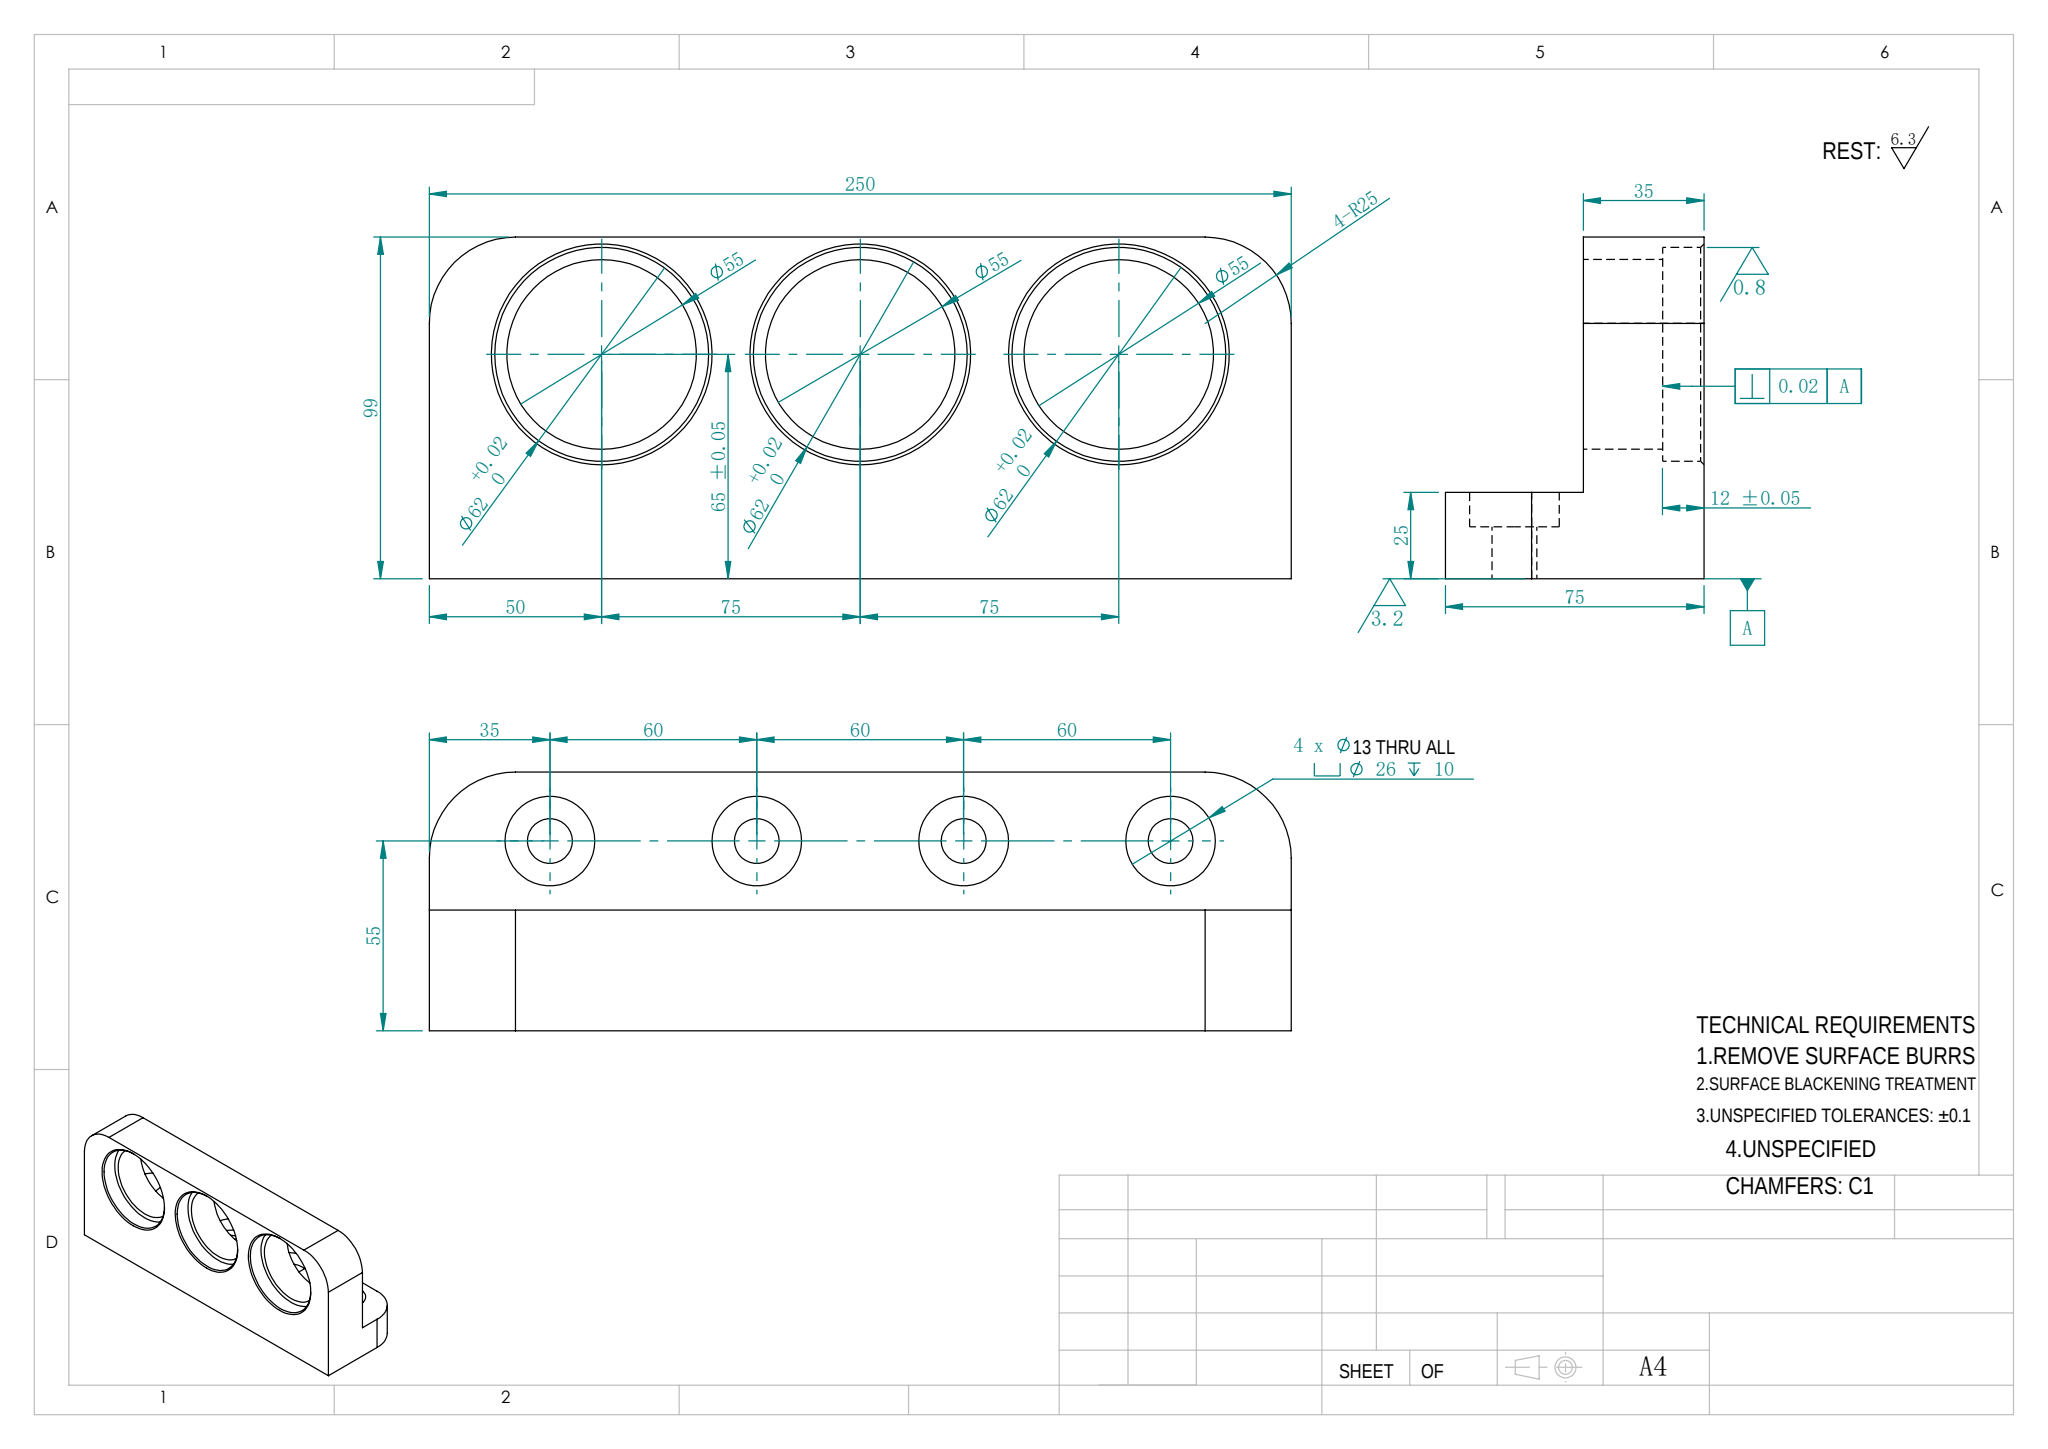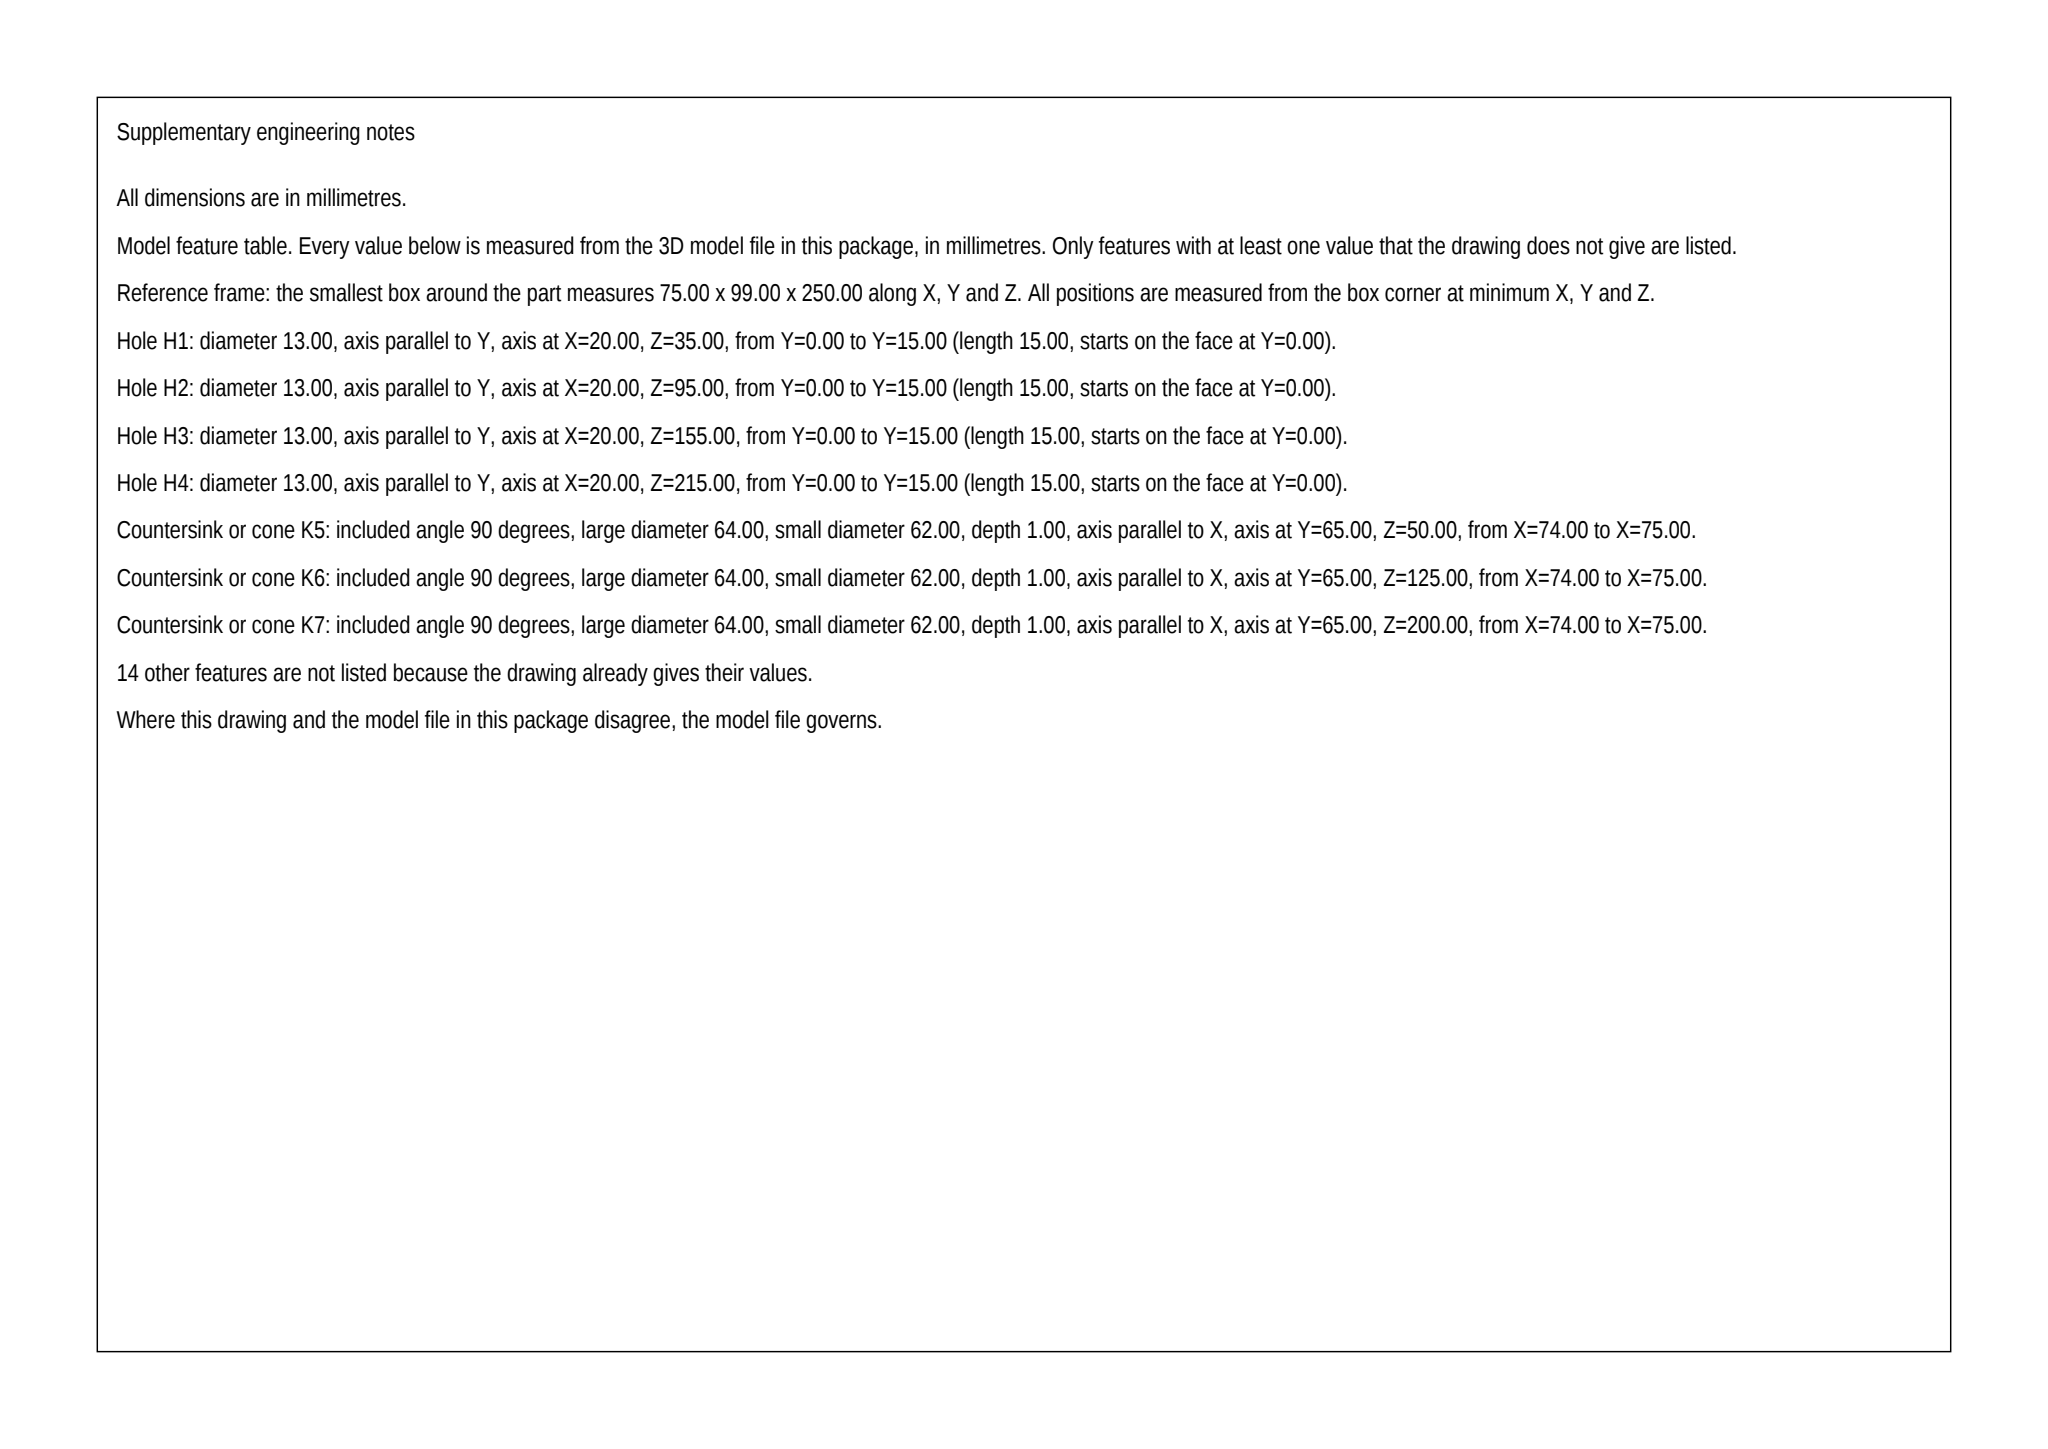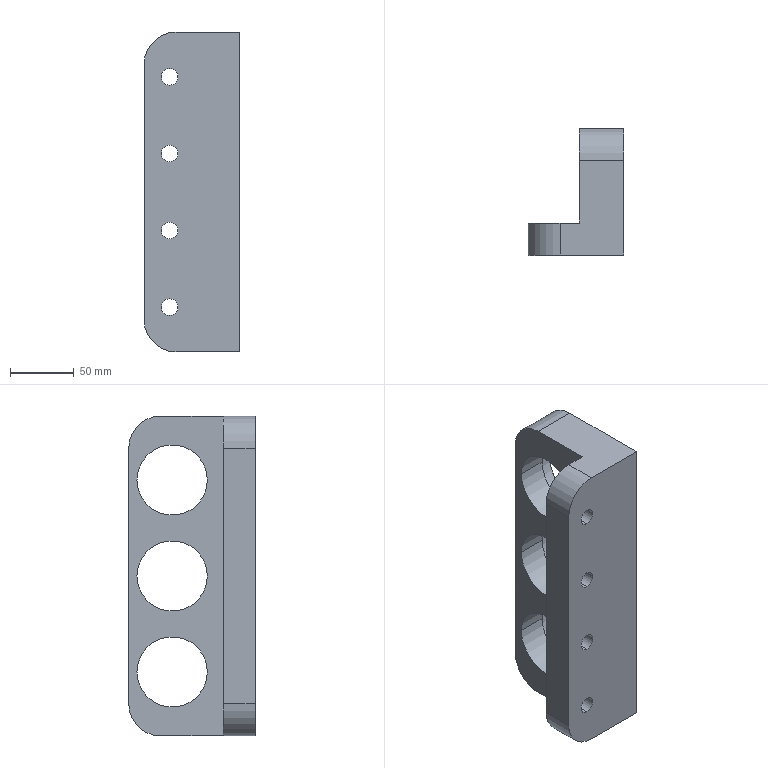Part | SolidWorks | mm | 1 solid | 53 faces | box 75 x 99 x 250 mm | volume 798040 mm3 | cylinder 32 | plane 15 | cone 6 | commonest cylinder face diameters 26 x8 13 x8 55 x6 62 x6 50 x4
build123d program:
from build123d import *

# Parameters (mm, degrees)
BOSS_EXTRUDE1_DEPTH                                  = 250
SKETCH2_R                                            = 31
CUT_EXTRUDE1_DEPTH                                   = 12
CYLINDRICAL_COUNTERSUNK_HOLE_FOR_M12_HEX_D           = 13
CYLINDRICAL_COUNTERSUNK_HOLE_FOR_M12_HEX_CBORE_D     = 26
CYLINDRICAL_COUNTERSUNK_HOLE_FOR_M12_HEX_CBORE_DEPTH = 10
FILLET1_R                                            = 25
SKETCH9_R                                            = 27.5
CUT_EXTRUDE2_DEPTH                                   = 269.226
CHAMFER1_SIZE                                        = 1


with BuildPart() as part:
    # Sketch1 → Boss-Extrude1 (new body)
    with BuildSketch(Plane.XY):
        Polygon((0, 74), (0, 0), (-40, 0), (-40, -25), (35, -25), (35, 74), align=None)
    extrude(amount=BOSS_EXTRUDE1_DEPTH)

    # Sketch2 → Cut-Extrude1 (cut)
    with BuildSketch(Plane(origin=(35, 0, 0), x_dir=(0, 0, -1), z_dir=(1, 0, 0))):
        with Locations(Location((-200, 40, 0), (0, 0, 90))):
            Circle(SKETCH2_R)
        with Locations(Location((-125, 40, 0), (0, 0, 90))):
            Circle(SKETCH2_R)
        with Locations(Location((-50, 40, 0), (0, 0, 90))):
            Circle(SKETCH2_R)
    extrude(amount=-CUT_EXTRUDE1_DEPTH, mode=Mode.SUBTRACT)

    # Cylindrical Countersunk Hole for M12 Hex (through all)
    with Locations(Plane(origin=(0, 0, 0), x_dir=(1, 0, 0), z_dir=(0, 1, 0))):
        with Locations((-20, -215), (-20, -155), (-20, -95), (-20, -35)):
            CounterBoreHole(CYLINDRICAL_COUNTERSUNK_HOLE_FOR_M12_HEX_D / 2, CYLINDRICAL_COUNTERSUNK_HOLE_FOR_M12_HEX_CBORE_D / 2, CYLINDRICAL_COUNTERSUNK_HOLE_FOR_M12_HEX_CBORE_DEPTH)

    # Fillet1
    fillet1_edges = [part.edges().sort_by_distance(p)[0] for p in [
        (-40, -12.5, 250),
        (17.5, 74, 250),
        (-40, -12.5, 0),
        (17.5, 74, 0),
    ]]
    fillet(fillet1_edges, radius=FILLET1_R)

    # Sketch9 → Cut-Extrude2 (cut, through all)
    with BuildSketch(Plane(origin=(23, 0, 0), x_dir=(0, 0, -1), z_dir=(1, 0, 0))):
        with Locations(Location((-200, 40, 0), (0, 0, 90))):
            Circle(SKETCH9_R)
        with Locations(Location((-125, 40, 0), (0, 0, 90))):
            Circle(SKETCH9_R)
        with Locations(Location((-50, 40, 0), (0, 0, 90))):
            Circle(SKETCH9_R)
    extrude(amount=-CUT_EXTRUDE2_DEPTH, mode=Mode.SUBTRACT)

    # Chamfer1
    chamfer1_edges = [part.edges().sort_by_distance(p)[0] for p in [
        (35, 9, 200),
        (35, 9, 125),
        (35, 9, 50),
    ]]
    chamfer(chamfer1_edges, length=CHAMFER1_SIZE)


solid = part.part